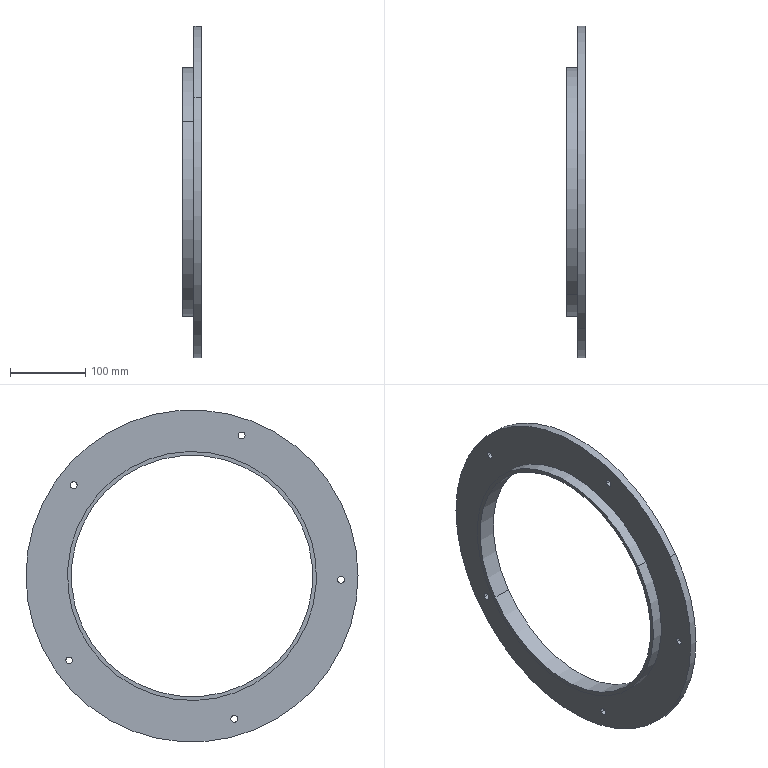Component | SolidWorks | SeedingAssemblyA-1_SeedingFixingPlateA-1 | 1 solid | 19 faces | box 25 x 440 x 440 mm | volume 789679 mm3 | cylinder 16 | plane 3 | commonest cylinder face diameters 9 x10 320 x2 330 x2 440 x2
STEP:
#1=COLOUR_RGB('',0.7922,0.8196,0.9333);
#2=FILL_AREA_STYLE_COLOUR('',#1);
#3=FILL_AREA_STYLE('',(#2));
#4=SURFACE_STYLE_FILL_AREA(#3);
#5=SURFACE_SIDE_STYLE('',(#4));
#6=SURFACE_STYLE_USAGE(.BOTH.,#5);
#7=PRESENTATION_STYLE_ASSIGNMENT((#6));
#8=CARTESIAN_POINT('',(4.558,1.889,-5.094));
#9=VERTEX_POINT('',#8);
#10=CARTESIAN_POINT('',(4.558,2.181,-5.295));
#11=VERTEX_POINT('',#10);
#12=CARTESIAN_POINT('',(4.558,2.035,-5.195));
#13=DIRECTION('',(1.,-0.,-0.));
#14=DIRECTION('',(0.,0.8242,-0.5664));
#15=AXIS2_PLACEMENT_3D('',#12,#13,#14);
#16=CIRCLE('',#15,0.1772);
#17=EDGE_CURVE('',#9,#11,#16,.T.);
#18=ORIENTED_EDGE('',*,*,#17,.F.);
#19=CARTESIAN_POINT('',(4.952,1.889,-5.094));
#20=VERTEX_POINT('',#19);
#21=CARTESIAN_POINT('',(3.968,1.889,-5.094));
#22=DIRECTION('',(1.,-0.,-0.));
#23=VECTOR('',#22,39.37);
#24=LINE('',#21,#23);
#25=EDGE_CURVE('',#9,#20,#24,.T.);
#26=ORIENTED_EDGE('',*,*,#25,.T.);
#27=CARTESIAN_POINT('',(4.952,2.181,-5.295));
#28=VERTEX_POINT('',#27);
#29=CARTESIAN_POINT('',(4.952,2.035,-5.195));
#30=DIRECTION('',(1.,-0.,-0.));
#31=DIRECTION('',(0.,0.7933,0.6088));
#32=AXIS2_PLACEMENT_3D('',#29,#30,#31);
#33=CIRCLE('',#32,0.1772);
#34=EDGE_CURVE('',#20,#28,#33,.T.);
#35=ORIENTED_EDGE('',*,*,#34,.T.);
#36=CARTESIAN_POINT('',(3.968,2.181,-5.295));
#37=DIRECTION('',(1.,-0.,-0.));
#38=VECTOR('',#37,39.37);
#39=LINE('',#36,#38);
#40=EDGE_CURVE('',#11,#28,#39,.T.);
#41=ORIENTED_EDGE('',*,*,#40,.F.);
#42=EDGE_LOOP('',(#18,#26,#35,#41));
#43=FACE_OUTER_BOUND('',#42,.T.);
#44=CARTESIAN_POINT('',(3.968,2.035,-5.195));
#45=DIRECTION('',(1.,-0.,-0.));
#46=DIRECTION('',(0.,0.8242,-0.5664));
#47=AXIS2_PLACEMENT_3D('',#44,#45,#46);
#48=CYLINDRICAL_SURFACE('',#47,0.1772);
#49=ADVANCED_FACE('',(#43),#48,.F.);
#50=CARTESIAN_POINT('',(4.558,-6.876,-2.499));
#51=VERTEX_POINT('',#50);
#52=CARTESIAN_POINT('',(4.558,-6.584,-2.699));
#53=VERTEX_POINT('',#52);
#54=CARTESIAN_POINT('',(4.558,-6.73,-2.599));
#55=DIRECTION('',(1.,-0.,-0.));
#56=DIRECTION('',(0.,0.8242,-0.5664));
#57=AXIS2_PLACEMENT_3D('',#54,#55,#56);
#58=CIRCLE('',#57,0.1772);
#59=EDGE_CURVE('',#51,#53,#58,.T.);
#60=ORIENTED_EDGE('',*,*,#59,.F.);
#61=CARTESIAN_POINT('',(4.952,-6.876,-2.499));
#62=VERTEX_POINT('',#61);
#63=CARTESIAN_POINT('',(3.968,-6.876,-2.499));
#64=DIRECTION('',(1.,-0.,-0.));
#65=VECTOR('',#64,39.37);
#66=LINE('',#63,#65);
#67=EDGE_CURVE('',#51,#62,#66,.T.);
#68=ORIENTED_EDGE('',*,*,#67,.T.);
#69=CARTESIAN_POINT('',(4.952,-6.584,-2.699));
#70=VERTEX_POINT('',#69);
#71=CARTESIAN_POINT('',(4.952,-6.73,-2.599));
#72=DIRECTION('',(1.,-0.,-0.));
#73=DIRECTION('',(0.,-0.3339,0.9426));
#74=AXIS2_PLACEMENT_3D('',#71,#72,#73);
#75=CIRCLE('',#74,0.1772);
#76=EDGE_CURVE('',#62,#70,#75,.T.);
#77=ORIENTED_EDGE('',*,*,#76,.T.);
#78=CARTESIAN_POINT('',(3.968,-6.584,-2.699));
#79=DIRECTION('',(1.,-0.,-0.));
#80=VECTOR('',#79,39.37);
#81=LINE('',#78,#80);
#82=EDGE_CURVE('',#53,#70,#81,.T.);
#83=ORIENTED_EDGE('',*,*,#82,.F.);
#84=EDGE_LOOP('',(#60,#68,#77,#83));
#85=FACE_OUTER_BOUND('',#84,.T.);
#86=CARTESIAN_POINT('',(3.968,-6.73,-2.599));
#87=DIRECTION('',(1.,-0.,-0.));
#88=DIRECTION('',(0.,0.8242,-0.5664));
#89=AXIS2_PLACEMENT_3D('',#86,#87,#88);
#90=CYLINDRICAL_SURFACE('',#89,0.1772);
#91=ADVANCED_FACE('',(#85),#90,.F.);
#92=CARTESIAN_POINT('',(4.558,-12.053,-10.032));
#93=VERTEX_POINT('',#92);
#94=CARTESIAN_POINT('',(4.558,-11.761,-10.233));
#95=VERTEX_POINT('',#94);
#96=CARTESIAN_POINT('',(4.558,-11.907,-10.132));
#97=DIRECTION('',(1.,-0.,-0.));
#98=DIRECTION('',(0.,0.8242,-0.5664));
#99=AXIS2_PLACEMENT_3D('',#96,#97,#98);
#100=CIRCLE('',#99,0.1772);
#101=EDGE_CURVE('',#93,#95,#100,.T.);
#102=ORIENTED_EDGE('',*,*,#101,.F.);
#103=CARTESIAN_POINT('',(4.952,-12.053,-10.032));
#104=VERTEX_POINT('',#103);
#105=CARTESIAN_POINT('',(3.968,-12.053,-10.032));
#106=DIRECTION('',(1.,-0.,-0.));
#107=VECTOR('',#106,39.37);
#108=LINE('',#105,#107);
#109=EDGE_CURVE('',#93,#104,#108,.T.);
#110=ORIENTED_EDGE('',*,*,#109,.T.);
#111=CARTESIAN_POINT('',(4.952,-11.761,-10.233));
#112=VERTEX_POINT('',#111);
#113=CARTESIAN_POINT('',(4.952,-11.907,-10.132));
#114=DIRECTION('',(1.,-0.,-0.));
#115=DIRECTION('',(0.,-0.9997,-0.02624));
#116=AXIS2_PLACEMENT_3D('',#113,#114,#115);
#117=CIRCLE('',#116,0.1772);
#118=EDGE_CURVE('',#104,#112,#117,.T.);
#119=ORIENTED_EDGE('',*,*,#118,.T.);
#120=CARTESIAN_POINT('',(3.968,-11.761,-10.233));
#121=DIRECTION('',(1.,-0.,-0.));
#122=VECTOR('',#121,39.37);
#123=LINE('',#120,#122);
#124=EDGE_CURVE('',#95,#112,#123,.T.);
#125=ORIENTED_EDGE('',*,*,#124,.F.);
#126=EDGE_LOOP('',(#102,#110,#119,#125));
#127=FACE_OUTER_BOUND('',#126,.T.);
#128=CARTESIAN_POINT('',(3.968,-11.907,-10.132));
#129=DIRECTION('',(1.,-0.,-0.));
#130=DIRECTION('',(0.,0.8242,-0.5664));
#131=AXIS2_PLACEMENT_3D('',#128,#129,#130);
#132=CYLINDRICAL_SURFACE('',#131,0.1772);
#133=ADVANCED_FACE('',(#127),#132,.F.);
#134=CARTESIAN_POINT('',(4.558,-6.488,-17.284));
#135=VERTEX_POINT('',#134);
#136=CARTESIAN_POINT('',(4.558,-6.196,-17.484));
#137=VERTEX_POINT('',#136);
#138=CARTESIAN_POINT('',(4.558,-6.342,-17.384));
#139=DIRECTION('',(1.,-0.,-0.));
#140=DIRECTION('',(0.,0.8242,-0.5664));
#141=AXIS2_PLACEMENT_3D('',#138,#139,#140);
#142=CIRCLE('',#141,0.1772);
#143=EDGE_CURVE('',#135,#137,#142,.T.);
#144=ORIENTED_EDGE('',*,*,#143,.F.);
#145=CARTESIAN_POINT('',(4.952,-6.488,-17.284));
#146=VERTEX_POINT('',#145);
#147=CARTESIAN_POINT('',(3.968,-6.488,-17.284));
#148=DIRECTION('',(1.,-0.,-0.));
#149=VECTOR('',#148,39.37);
#150=LINE('',#147,#149);
#151=EDGE_CURVE('',#135,#146,#150,.T.);
#152=ORIENTED_EDGE('',*,*,#151,.T.);
#153=CARTESIAN_POINT('',(4.952,-6.196,-17.484));
#154=VERTEX_POINT('',#153);
#155=CARTESIAN_POINT('',(4.952,-6.342,-17.384));
#156=DIRECTION('',(1.,-0.,-0.));
#157=DIRECTION('',(0.,-0.284,-0.9588));
#158=AXIS2_PLACEMENT_3D('',#155,#156,#157);
#159=CIRCLE('',#158,0.1772);
#160=EDGE_CURVE('',#146,#154,#159,.T.);
#161=ORIENTED_EDGE('',*,*,#160,.T.);
#162=CARTESIAN_POINT('',(3.968,-6.196,-17.484));
#163=DIRECTION('',(1.,-0.,-0.));
#164=VECTOR('',#163,39.37);
#165=LINE('',#162,#164);
#166=EDGE_CURVE('',#137,#154,#165,.T.);
#167=ORIENTED_EDGE('',*,*,#166,.F.);
#168=EDGE_LOOP('',(#144,#152,#161,#167));
#169=FACE_OUTER_BOUND('',#168,.T.);
#170=CARTESIAN_POINT('',(3.968,-6.342,-17.384));
#171=DIRECTION('',(1.,-0.,-0.));
#172=DIRECTION('',(0.,0.8242,-0.5664));
#173=AXIS2_PLACEMENT_3D('',#170,#171,#172);
#174=CYLINDRICAL_SURFACE('',#173,0.1772);
#175=ADVANCED_FACE('',(#169),#174,.F.);
#176=CARTESIAN_POINT('',(4.558,2.128,-14.232));
#177=VERTEX_POINT('',#176);
#178=CARTESIAN_POINT('',(4.558,2.42,-14.433));
#179=VERTEX_POINT('',#178);
#180=CARTESIAN_POINT('',(4.558,2.274,-14.332));
#181=DIRECTION('',(1.,-0.,-0.));
#182=DIRECTION('',(0.,0.8242,-0.5664));
#183=AXIS2_PLACEMENT_3D('',#180,#181,#182);
#184=CIRCLE('',#183,0.1772);
#185=EDGE_CURVE('',#177,#179,#184,.T.);
#186=ORIENTED_EDGE('',*,*,#185,.F.);
#187=CARTESIAN_POINT('',(4.952,2.128,-14.232));
#188=VERTEX_POINT('',#187);
#189=CARTESIAN_POINT('',(3.968,2.128,-14.232));
#190=DIRECTION('',(1.,-0.,-0.));
#191=VECTOR('',#190,39.37);
#192=LINE('',#189,#191);
#193=EDGE_CURVE('',#177,#188,#192,.T.);
#194=ORIENTED_EDGE('',*,*,#193,.T.);
#195=CARTESIAN_POINT('',(4.952,2.42,-14.433));
#196=VERTEX_POINT('',#195);
#197=CARTESIAN_POINT('',(4.952,2.274,-14.332));
#198=DIRECTION('',(1.,-0.,-0.));
#199=DIRECTION('',(0.,0.8242,-0.5664));
#200=AXIS2_PLACEMENT_3D('',#197,#198,#199);
#201=CIRCLE('',#200,0.1772);
#202=EDGE_CURVE('',#188,#196,#201,.T.);
#203=ORIENTED_EDGE('',*,*,#202,.T.);
#204=CARTESIAN_POINT('',(3.968,2.42,-14.433));
#205=DIRECTION('',(1.,-0.,-0.));
#206=VECTOR('',#205,39.37);
#207=LINE('',#204,#206);
#208=EDGE_CURVE('',#179,#196,#207,.T.);
#209=ORIENTED_EDGE('',*,*,#208,.F.);
#210=EDGE_LOOP('',(#186,#194,#203,#209));
#211=FACE_OUTER_BOUND('',#210,.T.);
#212=CARTESIAN_POINT('',(3.968,2.274,-14.332));
#213=DIRECTION('',(1.,-0.,-0.));
#214=DIRECTION('',(0.,0.8242,-0.5664));
#215=AXIS2_PLACEMENT_3D('',#212,#213,#214);
#216=CYLINDRICAL_SURFACE('',#215,0.1772);
#217=ADVANCED_FACE('',(#211),#216,.F.);
#218=CARTESIAN_POINT('',(3.968,-9.325,-6.361));
#219=VERTEX_POINT('',#218);
#220=CARTESIAN_POINT('',(3.968,1.058,-13.496));
#221=VERTEX_POINT('',#220);
#222=CARTESIAN_POINT('',(3.968,-4.134,-9.928));
#223=DIRECTION('',(1.,-0.,-0.));
#224=DIRECTION('',(0.,0.8242,-0.5664));
#225=AXIS2_PLACEMENT_3D('',#222,#223,#224);
#226=CIRCLE('',#225,6.299);
#227=EDGE_CURVE('',#219,#221,#226,.T.);
#228=ORIENTED_EDGE('',*,*,#227,.F.);
#229=CARTESIAN_POINT('',(4.952,-9.325,-6.361));
#230=VERTEX_POINT('',#229);
#231=CARTESIAN_POINT('',(3.968,-9.325,-6.361));
#232=DIRECTION('',(1.,-0.,-0.));
#233=VECTOR('',#232,39.37);
#234=LINE('',#231,#233);
#235=EDGE_CURVE('',#219,#230,#234,.T.);
#236=ORIENTED_EDGE('',*,*,#235,.T.);
#237=CARTESIAN_POINT('',(4.952,1.058,-13.496));
#238=VERTEX_POINT('',#237);
#239=CARTESIAN_POINT('',(4.952,-4.134,-9.928));
#240=DIRECTION('',(1.,-0.,-0.));
#241=DIRECTION('',(0.,0.8242,-0.5664));
#242=AXIS2_PLACEMENT_3D('',#239,#240,#241);
#243=CIRCLE('',#242,6.299);
#244=EDGE_CURVE('',#230,#238,#243,.T.);
#245=ORIENTED_EDGE('',*,*,#244,.T.);
#246=CARTESIAN_POINT('',(3.968,1.058,-13.496));
#247=DIRECTION('',(1.,-0.,-0.));
#248=VECTOR('',#247,39.37);
#249=LINE('',#246,#248);
#250=EDGE_CURVE('',#221,#238,#249,.T.);
#251=ORIENTED_EDGE('',*,*,#250,.F.);
#252=EDGE_LOOP('',(#228,#236,#245,#251));
#253=FACE_OUTER_BOUND('',#252,.T.);
#254=CARTESIAN_POINT('',(3.968,-4.134,-9.928));
#255=DIRECTION('',(1.,-0.,-0.));
#256=DIRECTION('',(0.,0.8242,-0.5664));
#257=AXIS2_PLACEMENT_3D('',#254,#255,#256);
#258=CYLINDRICAL_SURFACE('',#257,6.299);
#259=ADVANCED_FACE('',(#253),#258,.F.);
#260=CARTESIAN_POINT('',(3.968,1.22,-13.608));
#261=VERTEX_POINT('',#260);
#262=CARTESIAN_POINT('',(3.968,-9.488,-6.249));
#263=VERTEX_POINT('',#262);
#264=CARTESIAN_POINT('',(3.968,-4.134,-9.928));
#265=DIRECTION('',(1.,-0.,-0.));
#266=DIRECTION('',(0.,0.8242,-0.5664));
#267=AXIS2_PLACEMENT_3D('',#264,#265,#266);
#268=CIRCLE('',#267,6.496);
#269=EDGE_CURVE('',#261,#263,#268,.T.);
#270=ORIENTED_EDGE('',*,*,#269,.T.);
#271=CARTESIAN_POINT('',(4.558,-9.488,-6.249));
#272=VERTEX_POINT('',#271);
#273=CARTESIAN_POINT('',(3.968,-9.488,-6.249));
#274=DIRECTION('',(1.,-0.,-0.));
#275=VECTOR('',#274,39.37);
#276=LINE('',#273,#275);
#277=EDGE_CURVE('',#263,#272,#276,.T.);
#278=ORIENTED_EDGE('',*,*,#277,.T.);
#279=CARTESIAN_POINT('',(4.558,1.22,-13.608));
#280=VERTEX_POINT('',#279);
#281=CARTESIAN_POINT('',(4.558,-4.134,-9.928));
#282=DIRECTION('',(1.,-0.,-0.));
#283=DIRECTION('',(0.,0.8242,-0.5664));
#284=AXIS2_PLACEMENT_3D('',#281,#282,#283);
#285=CIRCLE('',#284,6.496);
#286=EDGE_CURVE('',#280,#272,#285,.T.);
#287=ORIENTED_EDGE('',*,*,#286,.F.);
#288=CARTESIAN_POINT('',(3.968,1.22,-13.608));
#289=DIRECTION('',(1.,-0.,-0.));
#290=VECTOR('',#289,39.37);
#291=LINE('',#288,#290);
#292=EDGE_CURVE('',#261,#280,#291,.T.);
#293=ORIENTED_EDGE('',*,*,#292,.F.);
#294=EDGE_LOOP('',(#270,#278,#287,#293));
#295=FACE_OUTER_BOUND('',#294,.T.);
#296=CARTESIAN_POINT('',(3.968,-4.134,-9.928));
#297=DIRECTION('',(1.,-0.,-0.));
#298=DIRECTION('',(0.,0.8242,-0.5664));
#299=AXIS2_PLACEMENT_3D('',#296,#297,#298);
#300=CYLINDRICAL_SURFACE('',#299,6.496);
#301=ADVANCED_FACE('',(#295),#300,.T.);
#302=CARTESIAN_POINT('',(4.952,3.005,-14.834));
#303=VERTEX_POINT('',#302);
#304=CARTESIAN_POINT('',(4.952,-11.272,-5.023));
#305=VERTEX_POINT('',#304);
#306=CARTESIAN_POINT('',(4.952,-4.134,-9.928));
#307=DIRECTION('',(1.,-0.,-0.));
#308=DIRECTION('',(0.,0.8242,-0.5664));
#309=AXIS2_PLACEMENT_3D('',#306,#307,#308);
#310=CIRCLE('',#309,8.661);
#311=EDGE_CURVE('',#303,#305,#310,.T.);
#312=ORIENTED_EDGE('',*,*,#311,.F.);
#313=CARTESIAN_POINT('',(4.558,3.005,-14.834));
#314=VERTEX_POINT('',#313);
#315=CARTESIAN_POINT('',(4.952,3.005,-14.834));
#316=DIRECTION('',(-1.,0.,0.));
#317=VECTOR('',#316,39.37);
#318=LINE('',#315,#317);
#319=EDGE_CURVE('',#303,#314,#318,.T.);
#320=ORIENTED_EDGE('',*,*,#319,.T.);
#321=CARTESIAN_POINT('',(4.558,-11.272,-5.023));
#322=VERTEX_POINT('',#321);
#323=CARTESIAN_POINT('',(4.558,-4.134,-9.928));
#324=DIRECTION('',(1.,-0.,-0.));
#325=DIRECTION('',(0.,0.8242,-0.5664));
#326=AXIS2_PLACEMENT_3D('',#323,#324,#325);
#327=CIRCLE('',#326,8.661);
#328=EDGE_CURVE('',#314,#322,#327,.T.);
#329=ORIENTED_EDGE('',*,*,#328,.T.);
#330=CARTESIAN_POINT('',(4.952,-11.272,-5.023));
#331=DIRECTION('',(-1.,0.,0.));
#332=VECTOR('',#331,39.37);
#333=LINE('',#330,#332);
#334=EDGE_CURVE('',#305,#322,#333,.T.);
#335=ORIENTED_EDGE('',*,*,#334,.F.);
#336=EDGE_LOOP('',(#312,#320,#329,#335));
#337=FACE_OUTER_BOUND('',#336,.T.);
#338=CARTESIAN_POINT('',(4.952,-4.134,-9.928));
#339=DIRECTION('',(-1.,0.,0.));
#340=DIRECTION('',(0.,-0.8242,0.5664));
#341=AXIS2_PLACEMENT_3D('',#338,#339,#340);
#342=CYLINDRICAL_SURFACE('',#341,8.661);
#343=ADVANCED_FACE('',(#337),#342,.T.);
#344=CARTESIAN_POINT('',(4.952,2.035,-5.195));
#345=DIRECTION('',(1.,-0.,-0.));
#346=DIRECTION('',(0.,0.7933,0.6088));
#347=AXIS2_PLACEMENT_3D('',#344,#345,#346);
#348=CIRCLE('',#347,0.1772);
#349=EDGE_CURVE('',#28,#20,#348,.T.);
#350=ORIENTED_EDGE('',*,*,#349,.F.);
#351=ORIENTED_EDGE('',*,*,#34,.F.);
#352=EDGE_LOOP('',(#350,#351));
#353=FACE_BOUND('',#352,.T.);
#354=CARTESIAN_POINT('',(4.952,-6.73,-2.599));
#355=DIRECTION('',(1.,-0.,-0.));
#356=DIRECTION('',(0.,-0.3339,0.9426));
#357=AXIS2_PLACEMENT_3D('',#354,#355,#356);
#358=CIRCLE('',#357,0.1772);
#359=EDGE_CURVE('',#70,#62,#358,.T.);
#360=ORIENTED_EDGE('',*,*,#359,.F.);
#361=ORIENTED_EDGE('',*,*,#76,.F.);
#362=EDGE_LOOP('',(#360,#361));
#363=FACE_BOUND('',#362,.T.);
#364=CARTESIAN_POINT('',(4.952,-11.907,-10.132));
#365=DIRECTION('',(1.,-0.,-0.));
#366=DIRECTION('',(0.,-0.9997,-0.02624));
#367=AXIS2_PLACEMENT_3D('',#364,#365,#366);
#368=CIRCLE('',#367,0.1772);
#369=EDGE_CURVE('',#112,#104,#368,.T.);
#370=ORIENTED_EDGE('',*,*,#369,.F.);
#371=ORIENTED_EDGE('',*,*,#118,.F.);
#372=EDGE_LOOP('',(#370,#371));
#373=FACE_BOUND('',#372,.T.);
#374=CARTESIAN_POINT('',(4.952,-6.342,-17.384));
#375=DIRECTION('',(1.,-0.,-0.));
#376=DIRECTION('',(0.,-0.284,-0.9588));
#377=AXIS2_PLACEMENT_3D('',#374,#375,#376);
#378=CIRCLE('',#377,0.1772);
#379=EDGE_CURVE('',#154,#146,#378,.T.);
#380=ORIENTED_EDGE('',*,*,#379,.F.);
#381=ORIENTED_EDGE('',*,*,#160,.F.);
#382=EDGE_LOOP('',(#380,#381));
#383=FACE_BOUND('',#382,.T.);
#384=CARTESIAN_POINT('',(4.952,2.274,-14.332));
#385=DIRECTION('',(1.,-0.,-0.));
#386=DIRECTION('',(0.,0.8242,-0.5664));
#387=AXIS2_PLACEMENT_3D('',#384,#385,#386);
#388=CIRCLE('',#387,0.1772);
#389=EDGE_CURVE('',#196,#188,#388,.T.);
#390=ORIENTED_EDGE('',*,*,#389,.F.);
#391=ORIENTED_EDGE('',*,*,#202,.F.);
#392=EDGE_LOOP('',(#390,#391));
#393=FACE_BOUND('',#392,.T.);
#394=CARTESIAN_POINT('',(4.952,-4.134,-9.928));
#395=DIRECTION('',(1.,-0.,-0.));
#396=DIRECTION('',(0.,0.8242,-0.5664));
#397=AXIS2_PLACEMENT_3D('',#394,#395,#396);
#398=CIRCLE('',#397,8.661);
#399=EDGE_CURVE('',#305,#303,#398,.T.);
#400=ORIENTED_EDGE('',*,*,#399,.T.);
#401=ORIENTED_EDGE('',*,*,#311,.T.);
#402=EDGE_LOOP('',(#400,#401));
#403=FACE_OUTER_BOUND('',#402,.T.);
#404=CARTESIAN_POINT('',(4.952,-4.134,-9.928));
#405=DIRECTION('',(1.,-0.,-0.));
#406=DIRECTION('',(0.,0.8242,-0.5664));
#407=AXIS2_PLACEMENT_3D('',#404,#405,#406);
#408=CIRCLE('',#407,6.299);
#409=EDGE_CURVE('',#238,#230,#408,.T.);
#410=ORIENTED_EDGE('',*,*,#409,.F.);
#411=ORIENTED_EDGE('',*,*,#244,.F.);
#412=EDGE_LOOP('',(#410,#411));
#413=FACE_BOUND('',#412,.T.);
#414=CARTESIAN_POINT('',(4.952,-4.134,-9.928));
#415=DIRECTION('',(1.,-0.,-0.));
#416=DIRECTION('',(0.,0.8242,-0.5664));
#417=AXIS2_PLACEMENT_3D('',#414,#415,#416);
#418=PLANE('',#417);
#419=ADVANCED_FACE('',(#353,#363,#373,#383,#393,#403,#413),#418,.T.);
#420=CARTESIAN_POINT('',(4.558,2.035,-5.195));
#421=DIRECTION('',(1.,-0.,-0.));
#422=DIRECTION('',(0.,0.8242,-0.5664));
#423=AXIS2_PLACEMENT_3D('',#420,#421,#422);
#424=CIRCLE('',#423,0.1772);
#425=EDGE_CURVE('',#11,#9,#424,.T.);
#426=ORIENTED_EDGE('',*,*,#425,.T.);
#427=ORIENTED_EDGE('',*,*,#17,.T.);
#428=EDGE_LOOP('',(#426,#427));
#429=FACE_BOUND('',#428,.T.);
#430=CARTESIAN_POINT('',(4.558,-6.73,-2.599));
#431=DIRECTION('',(1.,-0.,-0.));
#432=DIRECTION('',(0.,0.8242,-0.5664));
#433=AXIS2_PLACEMENT_3D('',#430,#431,#432);
#434=CIRCLE('',#433,0.1772);
#435=EDGE_CURVE('',#53,#51,#434,.T.);
#436=ORIENTED_EDGE('',*,*,#435,.T.);
#437=ORIENTED_EDGE('',*,*,#59,.T.);
#438=EDGE_LOOP('',(#436,#437));
#439=FACE_BOUND('',#438,.T.);
#440=CARTESIAN_POINT('',(4.558,-11.907,-10.132));
#441=DIRECTION('',(1.,-0.,-0.));
#442=DIRECTION('',(0.,0.8242,-0.5664));
#443=AXIS2_PLACEMENT_3D('',#440,#441,#442);
#444=CIRCLE('',#443,0.1772);
#445=EDGE_CURVE('',#95,#93,#444,.T.);
#446=ORIENTED_EDGE('',*,*,#445,.T.);
#447=ORIENTED_EDGE('',*,*,#101,.T.);
#448=EDGE_LOOP('',(#446,#447));
#449=FACE_BOUND('',#448,.T.);
#450=CARTESIAN_POINT('',(4.558,-6.342,-17.384));
#451=DIRECTION('',(1.,-0.,-0.));
#452=DIRECTION('',(0.,0.8242,-0.5664));
#453=AXIS2_PLACEMENT_3D('',#450,#451,#452);
#454=CIRCLE('',#453,0.1772);
#455=EDGE_CURVE('',#137,#135,#454,.T.);
#456=ORIENTED_EDGE('',*,*,#455,.T.);
#457=ORIENTED_EDGE('',*,*,#143,.T.);
#458=EDGE_LOOP('',(#456,#457));
#459=FACE_BOUND('',#458,.T.);
#460=CARTESIAN_POINT('',(4.558,2.274,-14.332));
#461=DIRECTION('',(1.,-0.,-0.));
#462=DIRECTION('',(0.,0.8242,-0.5664));
#463=AXIS2_PLACEMENT_3D('',#460,#461,#462);
#464=CIRCLE('',#463,0.1772);
#465=EDGE_CURVE('',#179,#177,#464,.T.);
#466=ORIENTED_EDGE('',*,*,#465,.T.);
#467=ORIENTED_EDGE('',*,*,#185,.T.);
#468=EDGE_LOOP('',(#466,#467));
#469=FACE_BOUND('',#468,.T.);
#470=CARTESIAN_POINT('',(4.558,-4.134,-9.928));
#471=DIRECTION('',(1.,-0.,-0.));
#472=DIRECTION('',(0.,0.8242,-0.5664));
#473=AXIS2_PLACEMENT_3D('',#470,#471,#472);
#474=CIRCLE('',#473,8.661);
#475=EDGE_CURVE('',#322,#314,#474,.T.);
#476=ORIENTED_EDGE('',*,*,#475,.F.);
#477=ORIENTED_EDGE('',*,*,#328,.F.);
#478=EDGE_LOOP('',(#476,#477));
#479=FACE_OUTER_BOUND('',#478,.T.);
#480=ORIENTED_EDGE('',*,*,#286,.T.);
#481=CARTESIAN_POINT('',(4.558,-4.134,-9.928));
#482=DIRECTION('',(1.,-0.,-0.));
#483=DIRECTION('',(0.,0.8242,-0.5664));
#484=AXIS2_PLACEMENT_3D('',#481,#482,#483);
#485=CIRCLE('',#484,6.496);
#486=EDGE_CURVE('',#272,#280,#485,.T.);
#487=ORIENTED_EDGE('',*,*,#486,.T.);
#488=EDGE_LOOP('',(#480,#487));
#489=FACE_BOUND('',#488,.T.);
#490=CARTESIAN_POINT('',(4.558,-4.134,-9.928));
#491=DIRECTION('',(1.,-0.,-0.));
#492=DIRECTION('',(0.,0.8242,-0.5664));
#493=AXIS2_PLACEMENT_3D('',#490,#491,#492);
#494=PLANE('',#493);
#495=ADVANCED_FACE('',(#429,#439,#449,#459,#469,#479,#489),#494,.F.);
#496=ORIENTED_EDGE('',*,*,#319,.F.);
#497=ORIENTED_EDGE('',*,*,#399,.F.);
#498=ORIENTED_EDGE('',*,*,#334,.T.);
#499=ORIENTED_EDGE('',*,*,#475,.T.);
#500=EDGE_LOOP('',(#496,#497,#498,#499));
#501=FACE_OUTER_BOUND('',#500,.T.);
#502=CARTESIAN_POINT('',(4.952,-4.134,-9.928));
#503=DIRECTION('',(-1.,0.,0.));
#504=DIRECTION('',(0.,-0.8242,0.5664));
#505=AXIS2_PLACEMENT_3D('',#502,#503,#504);
#506=CYLINDRICAL_SURFACE('',#505,8.661);
#507=ADVANCED_FACE('',(#501),#506,.T.);
#508=ORIENTED_EDGE('',*,*,#277,.F.);
#509=CARTESIAN_POINT('',(3.968,-4.134,-9.928));
#510=DIRECTION('',(1.,-0.,-0.));
#511=DIRECTION('',(0.,0.8242,-0.5664));
#512=AXIS2_PLACEMENT_3D('',#509,#510,#511);
#513=CIRCLE('',#512,6.496);
#514=EDGE_CURVE('',#263,#261,#513,.T.);
#515=ORIENTED_EDGE('',*,*,#514,.T.);
#516=ORIENTED_EDGE('',*,*,#292,.T.);
#517=ORIENTED_EDGE('',*,*,#486,.F.);
#518=EDGE_LOOP('',(#508,#515,#516,#517));
#519=FACE_OUTER_BOUND('',#518,.T.);
#520=CARTESIAN_POINT('',(3.968,-4.134,-9.928));
#521=DIRECTION('',(1.,-0.,-0.));
#522=DIRECTION('',(0.,0.8242,-0.5664));
#523=AXIS2_PLACEMENT_3D('',#520,#521,#522);
#524=CYLINDRICAL_SURFACE('',#523,6.496);
#525=ADVANCED_FACE('',(#519),#524,.T.);
#526=CARTESIAN_POINT('',(3.968,-4.134,-9.928));
#527=DIRECTION('',(1.,-0.,-0.));
#528=DIRECTION('',(0.,0.8242,-0.5664));
#529=AXIS2_PLACEMENT_3D('',#526,#527,#528);
#530=CIRCLE('',#529,6.299);
#531=EDGE_CURVE('',#221,#219,#530,.T.);
#532=ORIENTED_EDGE('',*,*,#531,.T.);
#533=ORIENTED_EDGE('',*,*,#227,.T.);
#534=EDGE_LOOP('',(#532,#533));
#535=FACE_BOUND('',#534,.T.);
#536=ORIENTED_EDGE('',*,*,#269,.F.);
#537=ORIENTED_EDGE('',*,*,#514,.F.);
#538=EDGE_LOOP('',(#536,#537));
#539=FACE_OUTER_BOUND('',#538,.T.);
#540=CARTESIAN_POINT('',(3.968,-4.134,-9.928));
#541=DIRECTION('',(1.,-0.,-0.));
#542=DIRECTION('',(0.,0.8242,-0.5664));
#543=AXIS2_PLACEMENT_3D('',#540,#541,#542);
#544=PLANE('',#543);
#545=ADVANCED_FACE('',(#535,#539),#544,.F.);
#546=ORIENTED_EDGE('',*,*,#235,.F.);
#547=ORIENTED_EDGE('',*,*,#531,.F.);
#548=ORIENTED_EDGE('',*,*,#250,.T.);
#549=ORIENTED_EDGE('',*,*,#409,.T.);
#550=EDGE_LOOP('',(#546,#547,#548,#549));
#551=FACE_OUTER_BOUND('',#550,.T.);
#552=CARTESIAN_POINT('',(3.968,-4.134,-9.928));
#553=DIRECTION('',(1.,-0.,-0.));
#554=DIRECTION('',(0.,0.8242,-0.5664));
#555=AXIS2_PLACEMENT_3D('',#552,#553,#554);
#556=CYLINDRICAL_SURFACE('',#555,6.299);
#557=ADVANCED_FACE('',(#551),#556,.F.);
#558=ORIENTED_EDGE('',*,*,#193,.F.);
#559=ORIENTED_EDGE('',*,*,#465,.F.);
#560=ORIENTED_EDGE('',*,*,#208,.T.);
#561=ORIENTED_EDGE('',*,*,#389,.T.);
#562=EDGE_LOOP('',(#558,#559,#560,#561));
#563=FACE_OUTER_BOUND('',#562,.T.);
#564=CARTESIAN_POINT('',(3.968,2.274,-14.332));
#565=DIRECTION('',(1.,-0.,-0.));
#566=DIRECTION('',(0.,0.8242,-0.5664));
#567=AXIS2_PLACEMENT_3D('',#564,#565,#566);
#568=CYLINDRICAL_SURFACE('',#567,0.1772);
#569=ADVANCED_FACE('',(#563),#568,.F.);
#570=ORIENTED_EDGE('',*,*,#151,.F.);
#571=ORIENTED_EDGE('',*,*,#455,.F.);
#572=ORIENTED_EDGE('',*,*,#166,.T.);
#573=ORIENTED_EDGE('',*,*,#379,.T.);
#574=EDGE_LOOP('',(#570,#571,#572,#573));
#575=FACE_OUTER_BOUND('',#574,.T.);
#576=CARTESIAN_POINT('',(3.968,-6.342,-17.384));
#577=DIRECTION('',(1.,-0.,-0.));
#578=DIRECTION('',(0.,0.8242,-0.5664));
#579=AXIS2_PLACEMENT_3D('',#576,#577,#578);
#580=CYLINDRICAL_SURFACE('',#579,0.1772);
#581=ADVANCED_FACE('',(#575),#580,.F.);
#582=ORIENTED_EDGE('',*,*,#109,.F.);
#583=ORIENTED_EDGE('',*,*,#445,.F.);
#584=ORIENTED_EDGE('',*,*,#124,.T.);
#585=ORIENTED_EDGE('',*,*,#369,.T.);
#586=EDGE_LOOP('',(#582,#583,#584,#585));
#587=FACE_OUTER_BOUND('',#586,.T.);
#588=CARTESIAN_POINT('',(3.968,-11.907,-10.132));
#589=DIRECTION('',(1.,-0.,-0.));
#590=DIRECTION('',(0.,0.8242,-0.5664));
#591=AXIS2_PLACEMENT_3D('',#588,#589,#590);
#592=CYLINDRICAL_SURFACE('',#591,0.1772);
#593=ADVANCED_FACE('',(#587),#592,.F.);
#594=ORIENTED_EDGE('',*,*,#67,.F.);
#595=ORIENTED_EDGE('',*,*,#435,.F.);
#596=ORIENTED_EDGE('',*,*,#82,.T.);
#597=ORIENTED_EDGE('',*,*,#359,.T.);
#598=EDGE_LOOP('',(#594,#595,#596,#597));
#599=FACE_OUTER_BOUND('',#598,.T.);
#600=CARTESIAN_POINT('',(3.968,-6.73,-2.599));
#601=DIRECTION('',(1.,-0.,-0.));
#602=DIRECTION('',(0.,0.8242,-0.5664));
#603=AXIS2_PLACEMENT_3D('',#600,#601,#602);
#604=CYLINDRICAL_SURFACE('',#603,0.1772);
#605=ADVANCED_FACE('',(#599),#604,.F.);
#606=ORIENTED_EDGE('',*,*,#25,.F.);
#607=ORIENTED_EDGE('',*,*,#425,.F.);
#608=ORIENTED_EDGE('',*,*,#40,.T.);
#609=ORIENTED_EDGE('',*,*,#349,.T.);
#610=EDGE_LOOP('',(#606,#607,#608,#609));
#611=FACE_OUTER_BOUND('',#610,.T.);
#612=CARTESIAN_POINT('',(3.968,2.035,-5.195));
#613=DIRECTION('',(1.,-0.,-0.));
#614=DIRECTION('',(0.,0.8242,-0.5664));
#615=AXIS2_PLACEMENT_3D('',#612,#613,#614);
#616=CYLINDRICAL_SURFACE('',#615,0.1772);
#617=ADVANCED_FACE('',(#611),#616,.F.);
#618=CLOSED_SHELL('',(#49,#91,#133,#175,#217,#259,#301,#343,#419,#495,#507,#525,#545,#557,#569,#581,#593,#605,#617));
#619=MANIFOLD_SOLID_BREP('',#618);
#620=STYLED_ITEM('',(#7),#619);
#621=(LENGTH_UNIT()NAMED_UNIT(*)SI_UNIT($,.METRE.));
#622=LENGTH_MEASURE_WITH_UNIT(LENGTH_MEASURE(0.0254),#621);
#623=DIMENSIONAL_EXPONENTS(1.,0.,0.,0.,0.,0.,0.);
#624=(CONVERSION_BASED_UNIT('',#622)LENGTH_UNIT()NAMED_UNIT(#623));
#625=UNCERTAINTY_MEASURE_WITH_UNIT(LENGTH_MEASURE(0.00001),#624,'','');
#626=(NAMED_UNIT(*)PLANE_ANGLE_UNIT()SI_UNIT($,.RADIAN.));
#627=(NAMED_UNIT(*)SI_UNIT($,.STERADIAN.)SOLID_ANGLE_UNIT());
#628=(GEOMETRIC_REPRESENTATION_CONTEXT(3)GLOBAL_UNCERTAINTY_ASSIGNED_CONTEXT((#625))GLOBAL_UNIT_ASSIGNED_CONTEXT((#624,#626,#627))REPRESENTATION_CONTEXT('',''));
#629=MECHANICAL_DESIGN_GEOMETRIC_PRESENTATION_REPRESENTATION('',(#620),#628);
#630=PRESENTATION_LAYER_ASSIGNMENT('','',(#620));
#631=CARTESIAN_POINT('',(0.,0.,0.));
#632=DIRECTION('',(0.,0.,1.));
#633=DIRECTION('',(1.,0.,0.));
#634=AXIS2_PLACEMENT_3D('',#631,#632,#633);
#635=(LENGTH_UNIT()NAMED_UNIT(*)SI_UNIT($,.METRE.));
#636=LENGTH_MEASURE_WITH_UNIT(LENGTH_MEASURE(0.0254),#635);
#637=DIMENSIONAL_EXPONENTS(1.,0.,0.,0.,0.,0.,0.);
#638=(CONVERSION_BASED_UNIT('',#636)LENGTH_UNIT()NAMED_UNIT(#637));
#639=UNCERTAINTY_MEASURE_WITH_UNIT(LENGTH_MEASURE(0.00001),#638,'','');
#640=(NAMED_UNIT(*)PLANE_ANGLE_UNIT()SI_UNIT($,.RADIAN.));
#641=(NAMED_UNIT(*)SI_UNIT($,.STERADIAN.)SOLID_ANGLE_UNIT());
#642=(GEOMETRIC_REPRESENTATION_CONTEXT(3)GLOBAL_UNCERTAINTY_ASSIGNED_CONTEXT((#639))GLOBAL_UNIT_ASSIGNED_CONTEXT((#638,#640,#641))REPRESENTATION_CONTEXT('',''));
#643=ADVANCED_BREP_SHAPE_REPRESENTATION('',(#619,#634),#642);